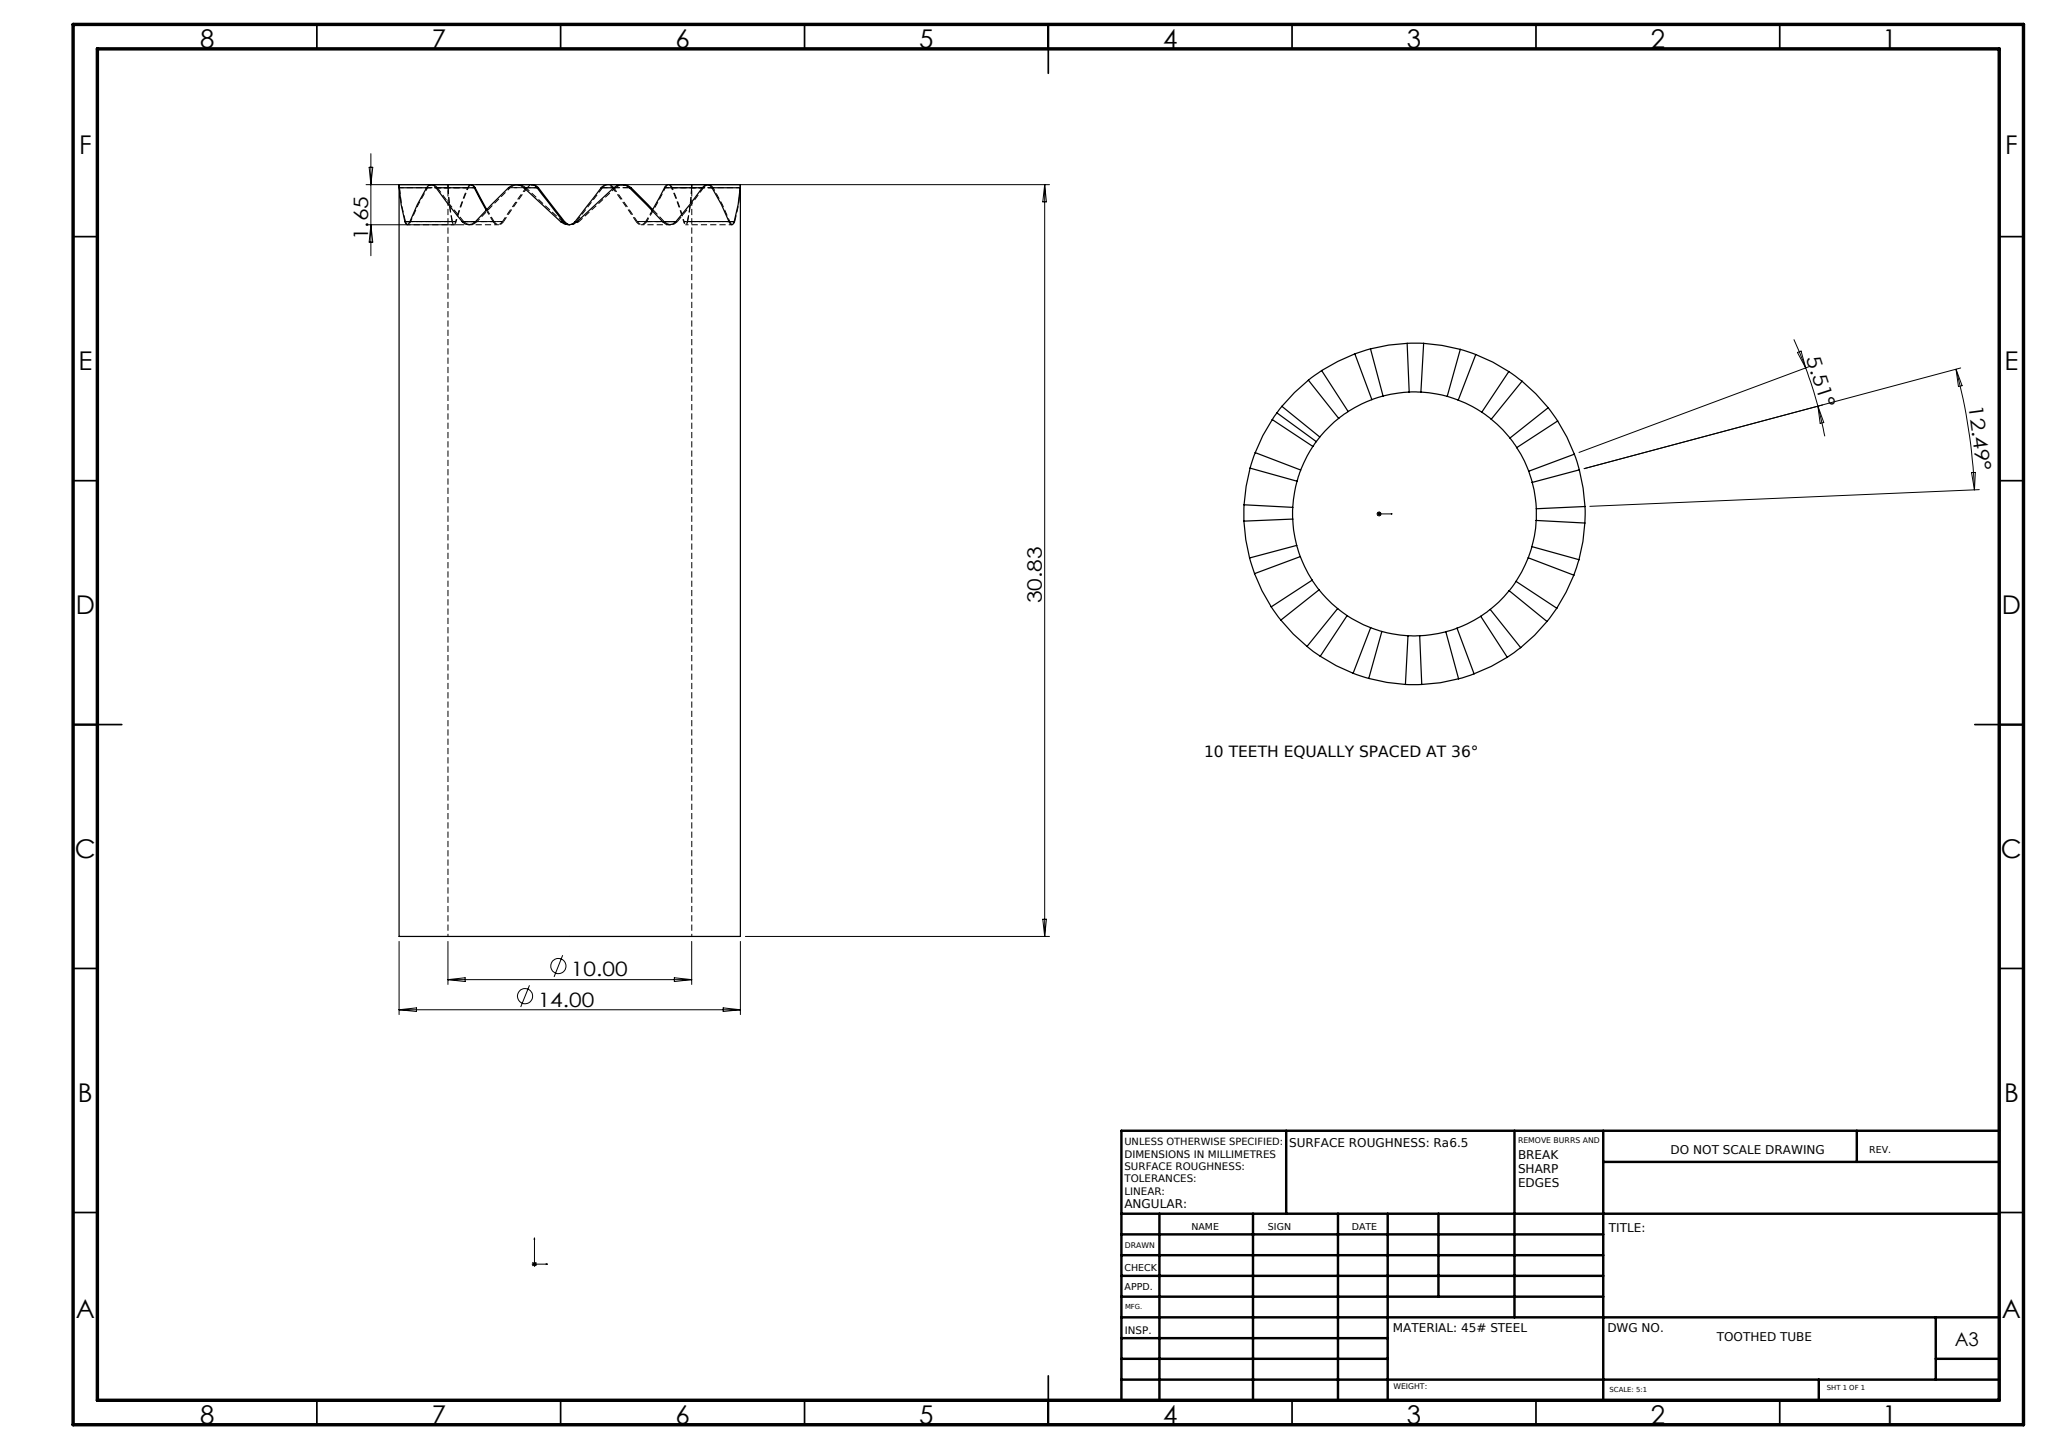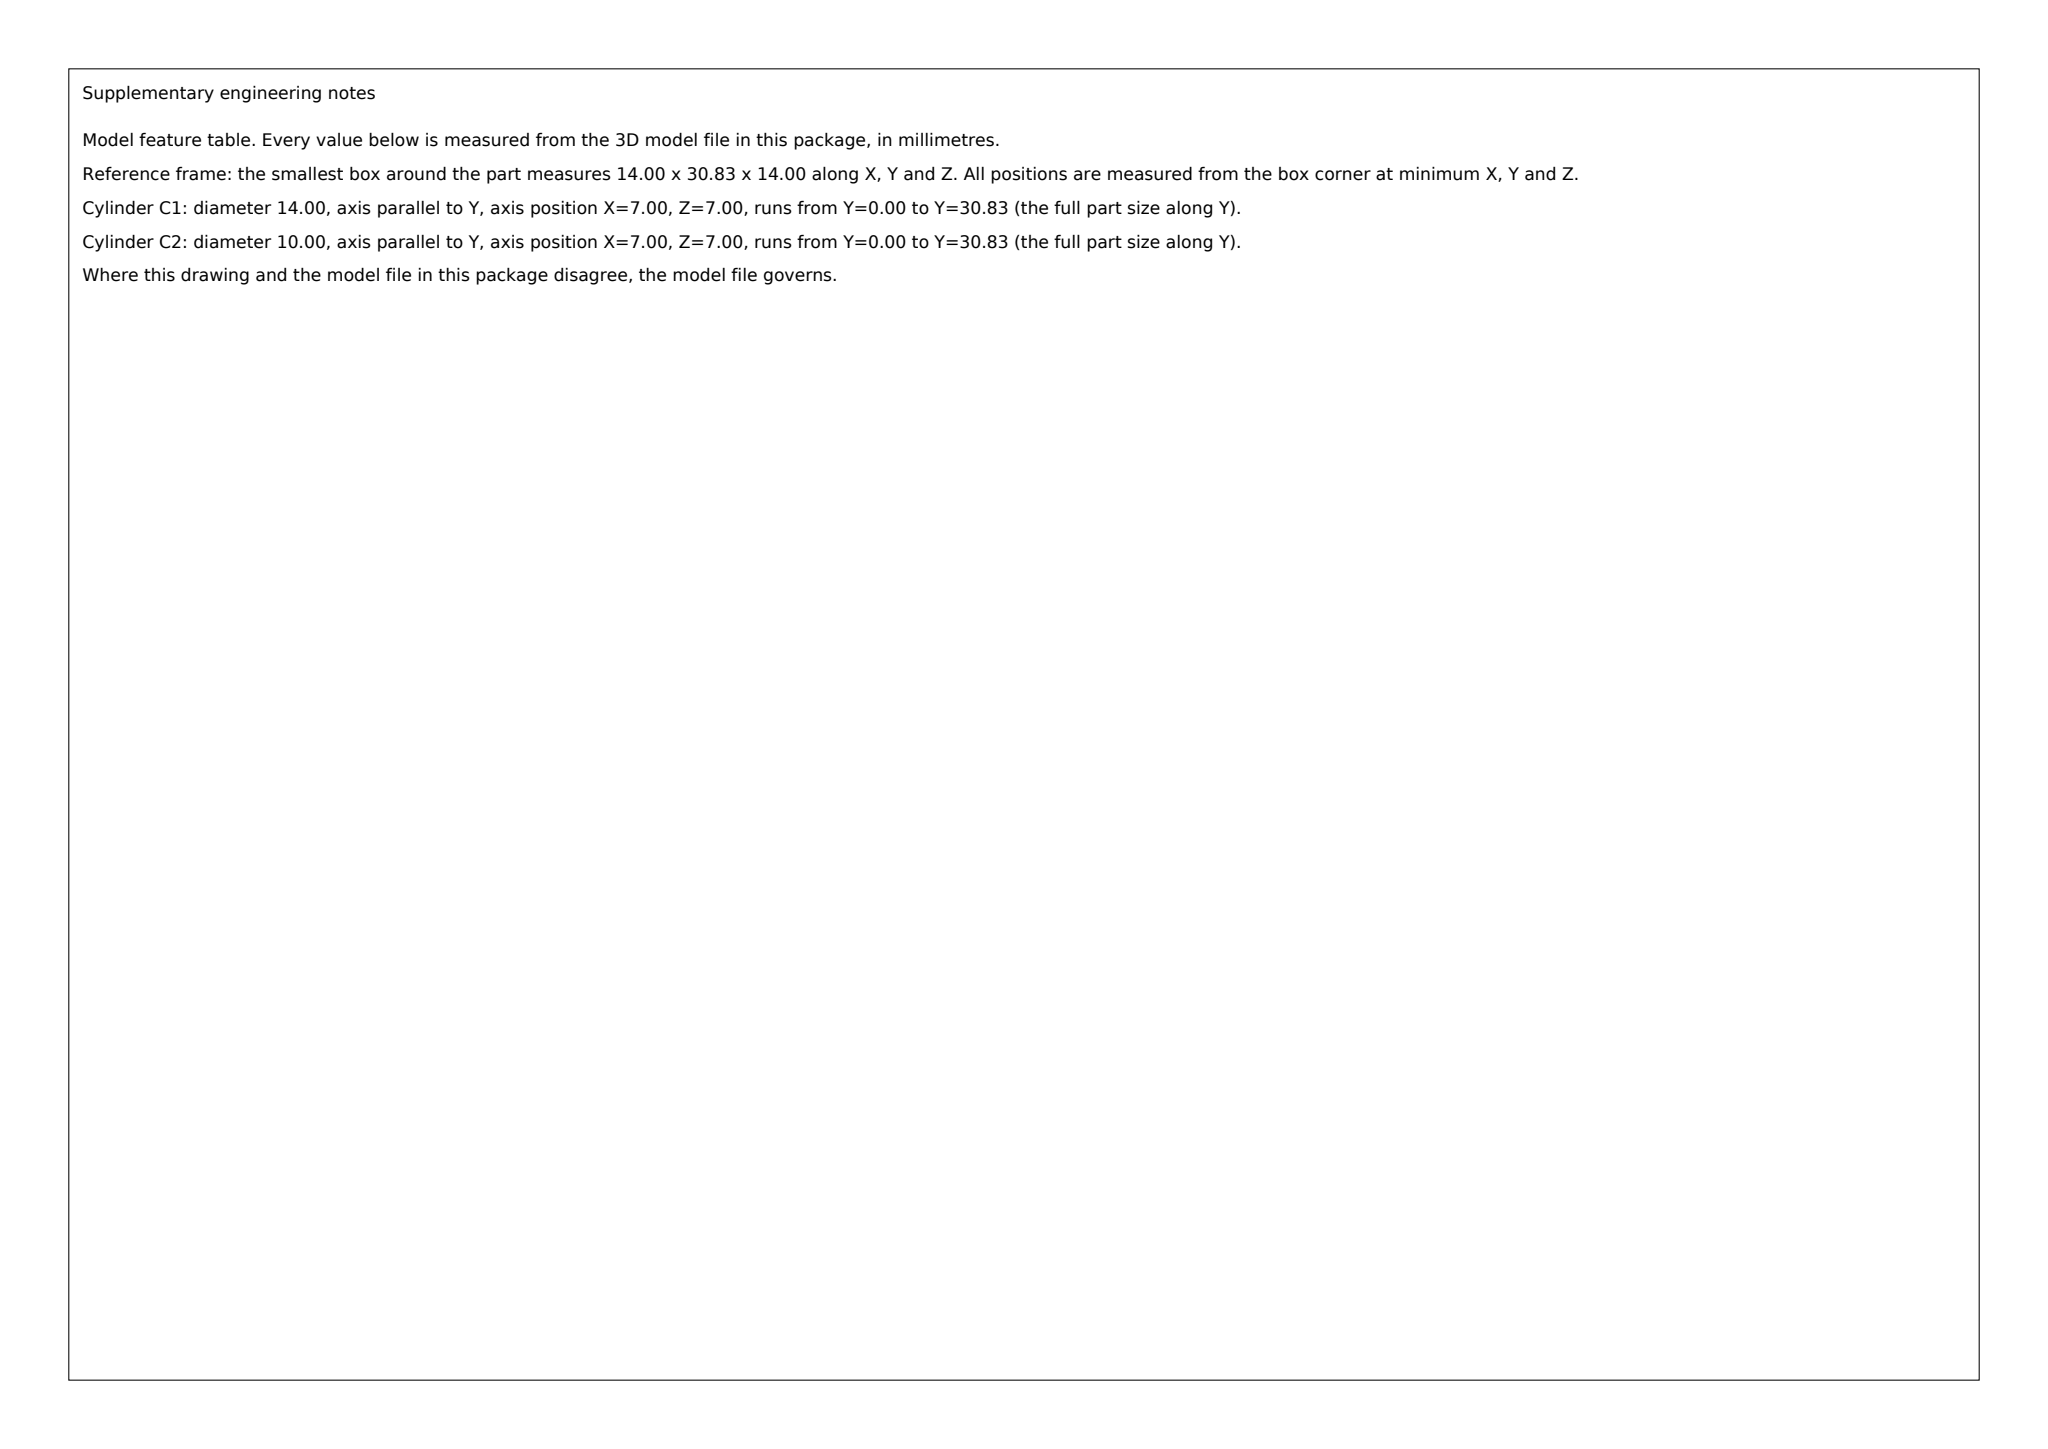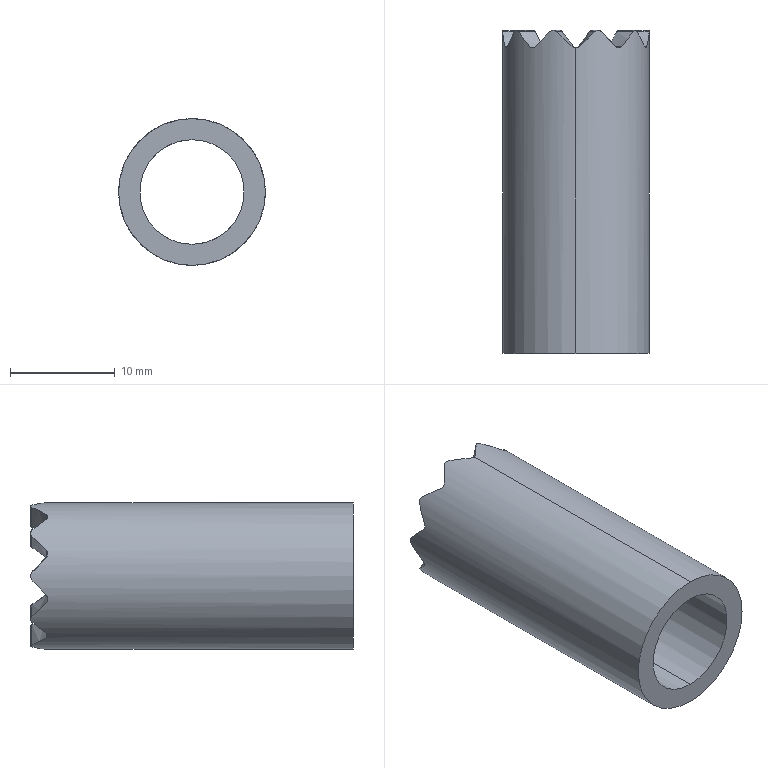Part | SolidWorks | mm | 1 solid | 46 faces | box 14 x 30.83 x 14 mm | volume 2262 mm3 | spline 41 | cylinder 4 | plane 1 | commonest cylinder face diameters 10 x2 14 x2